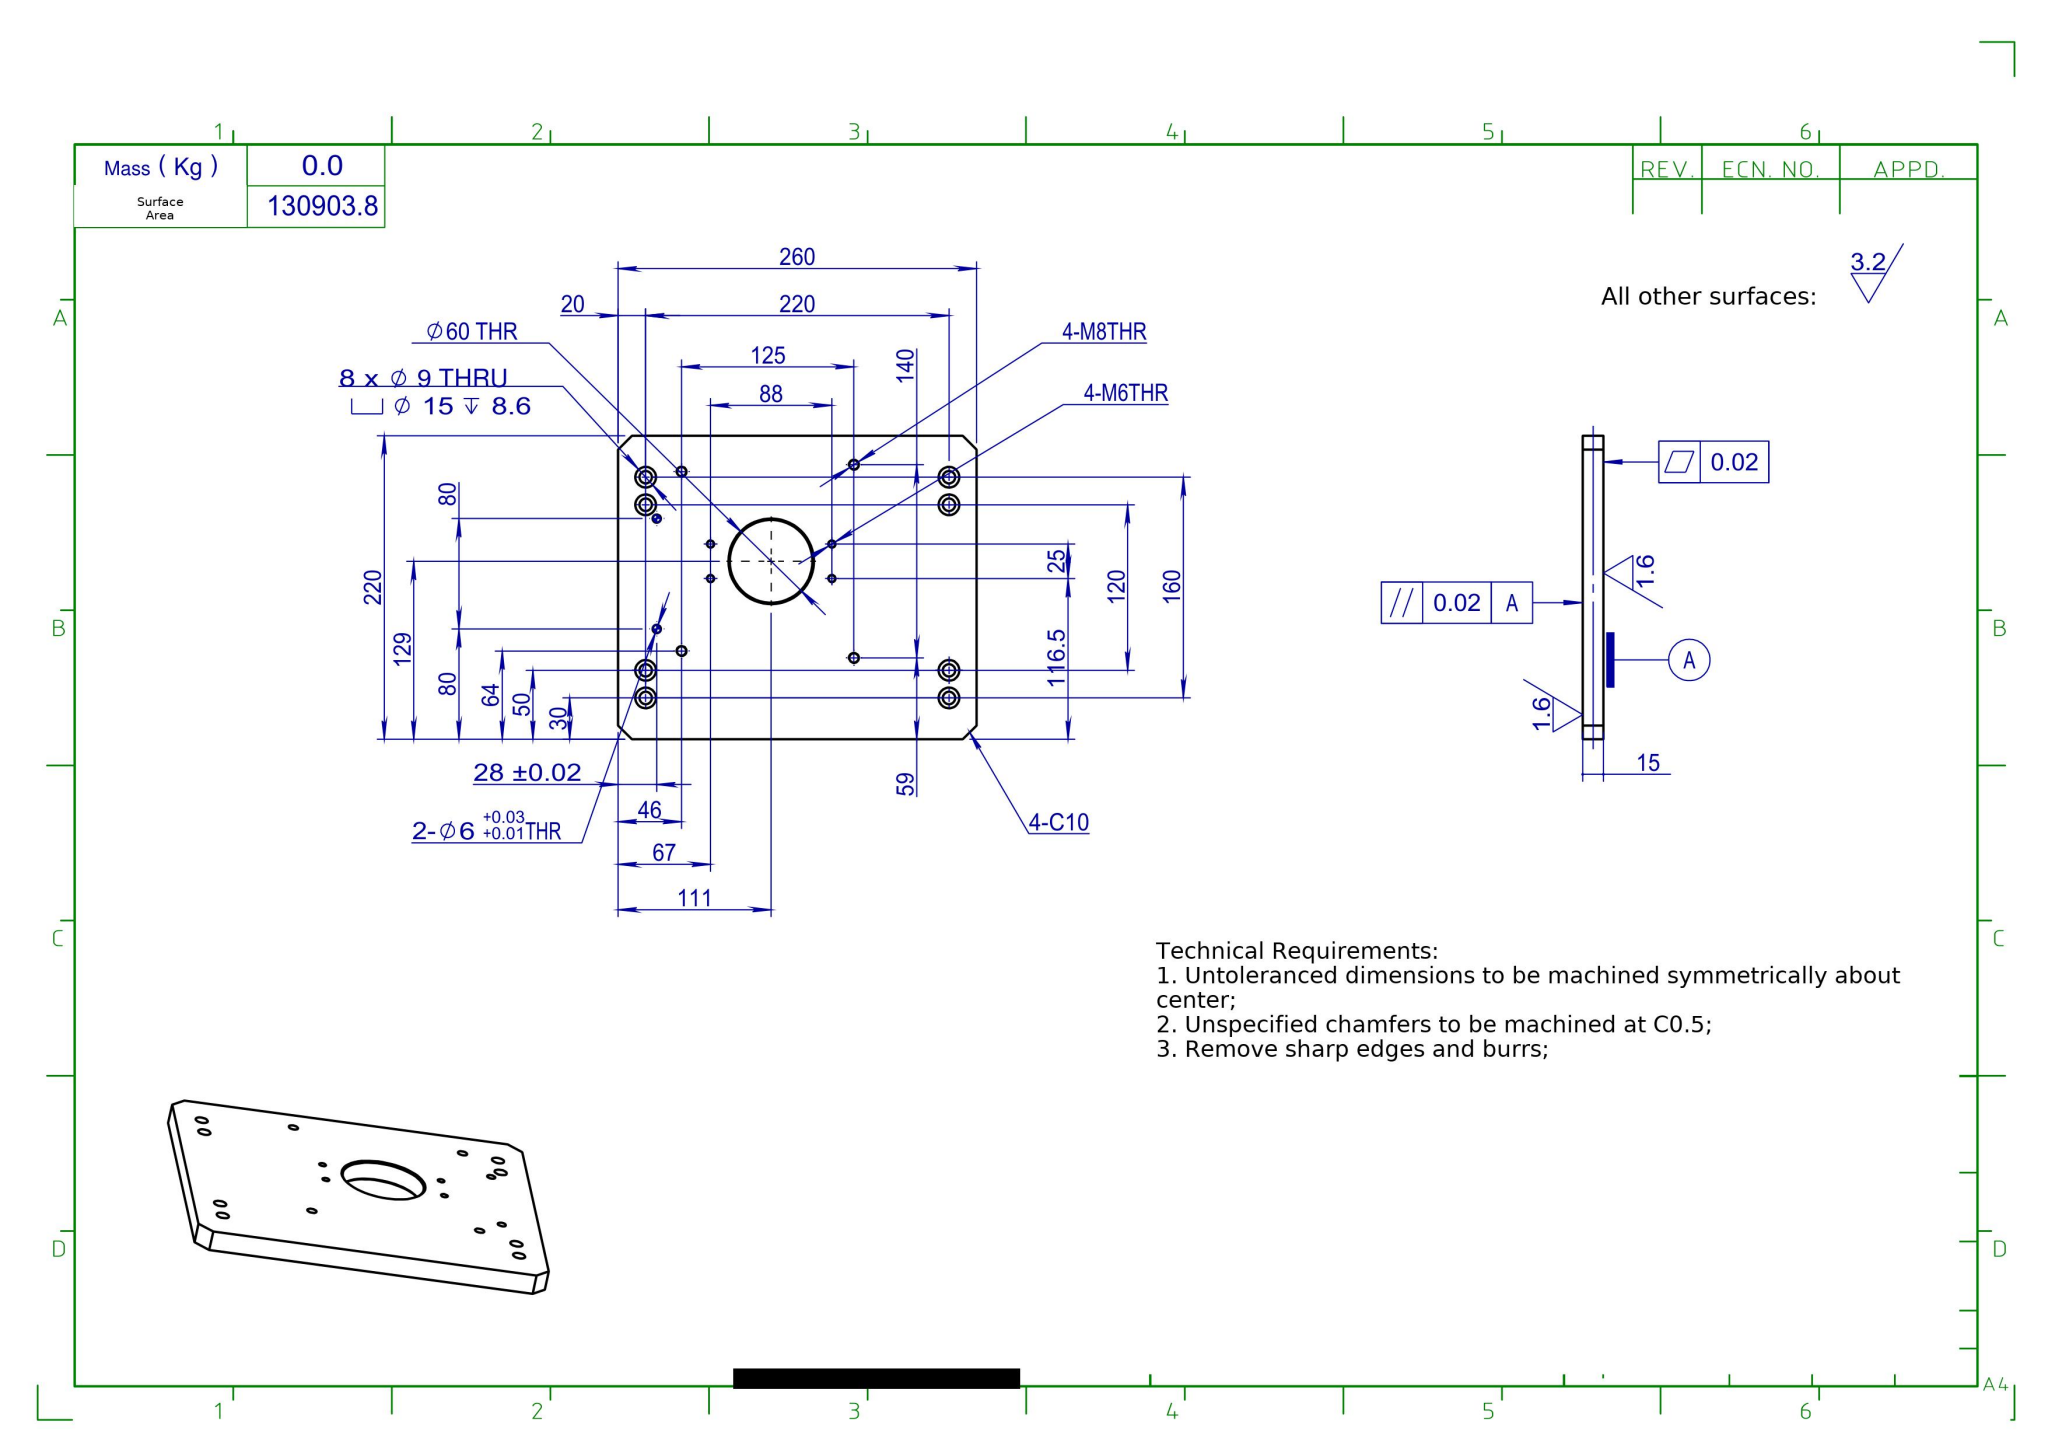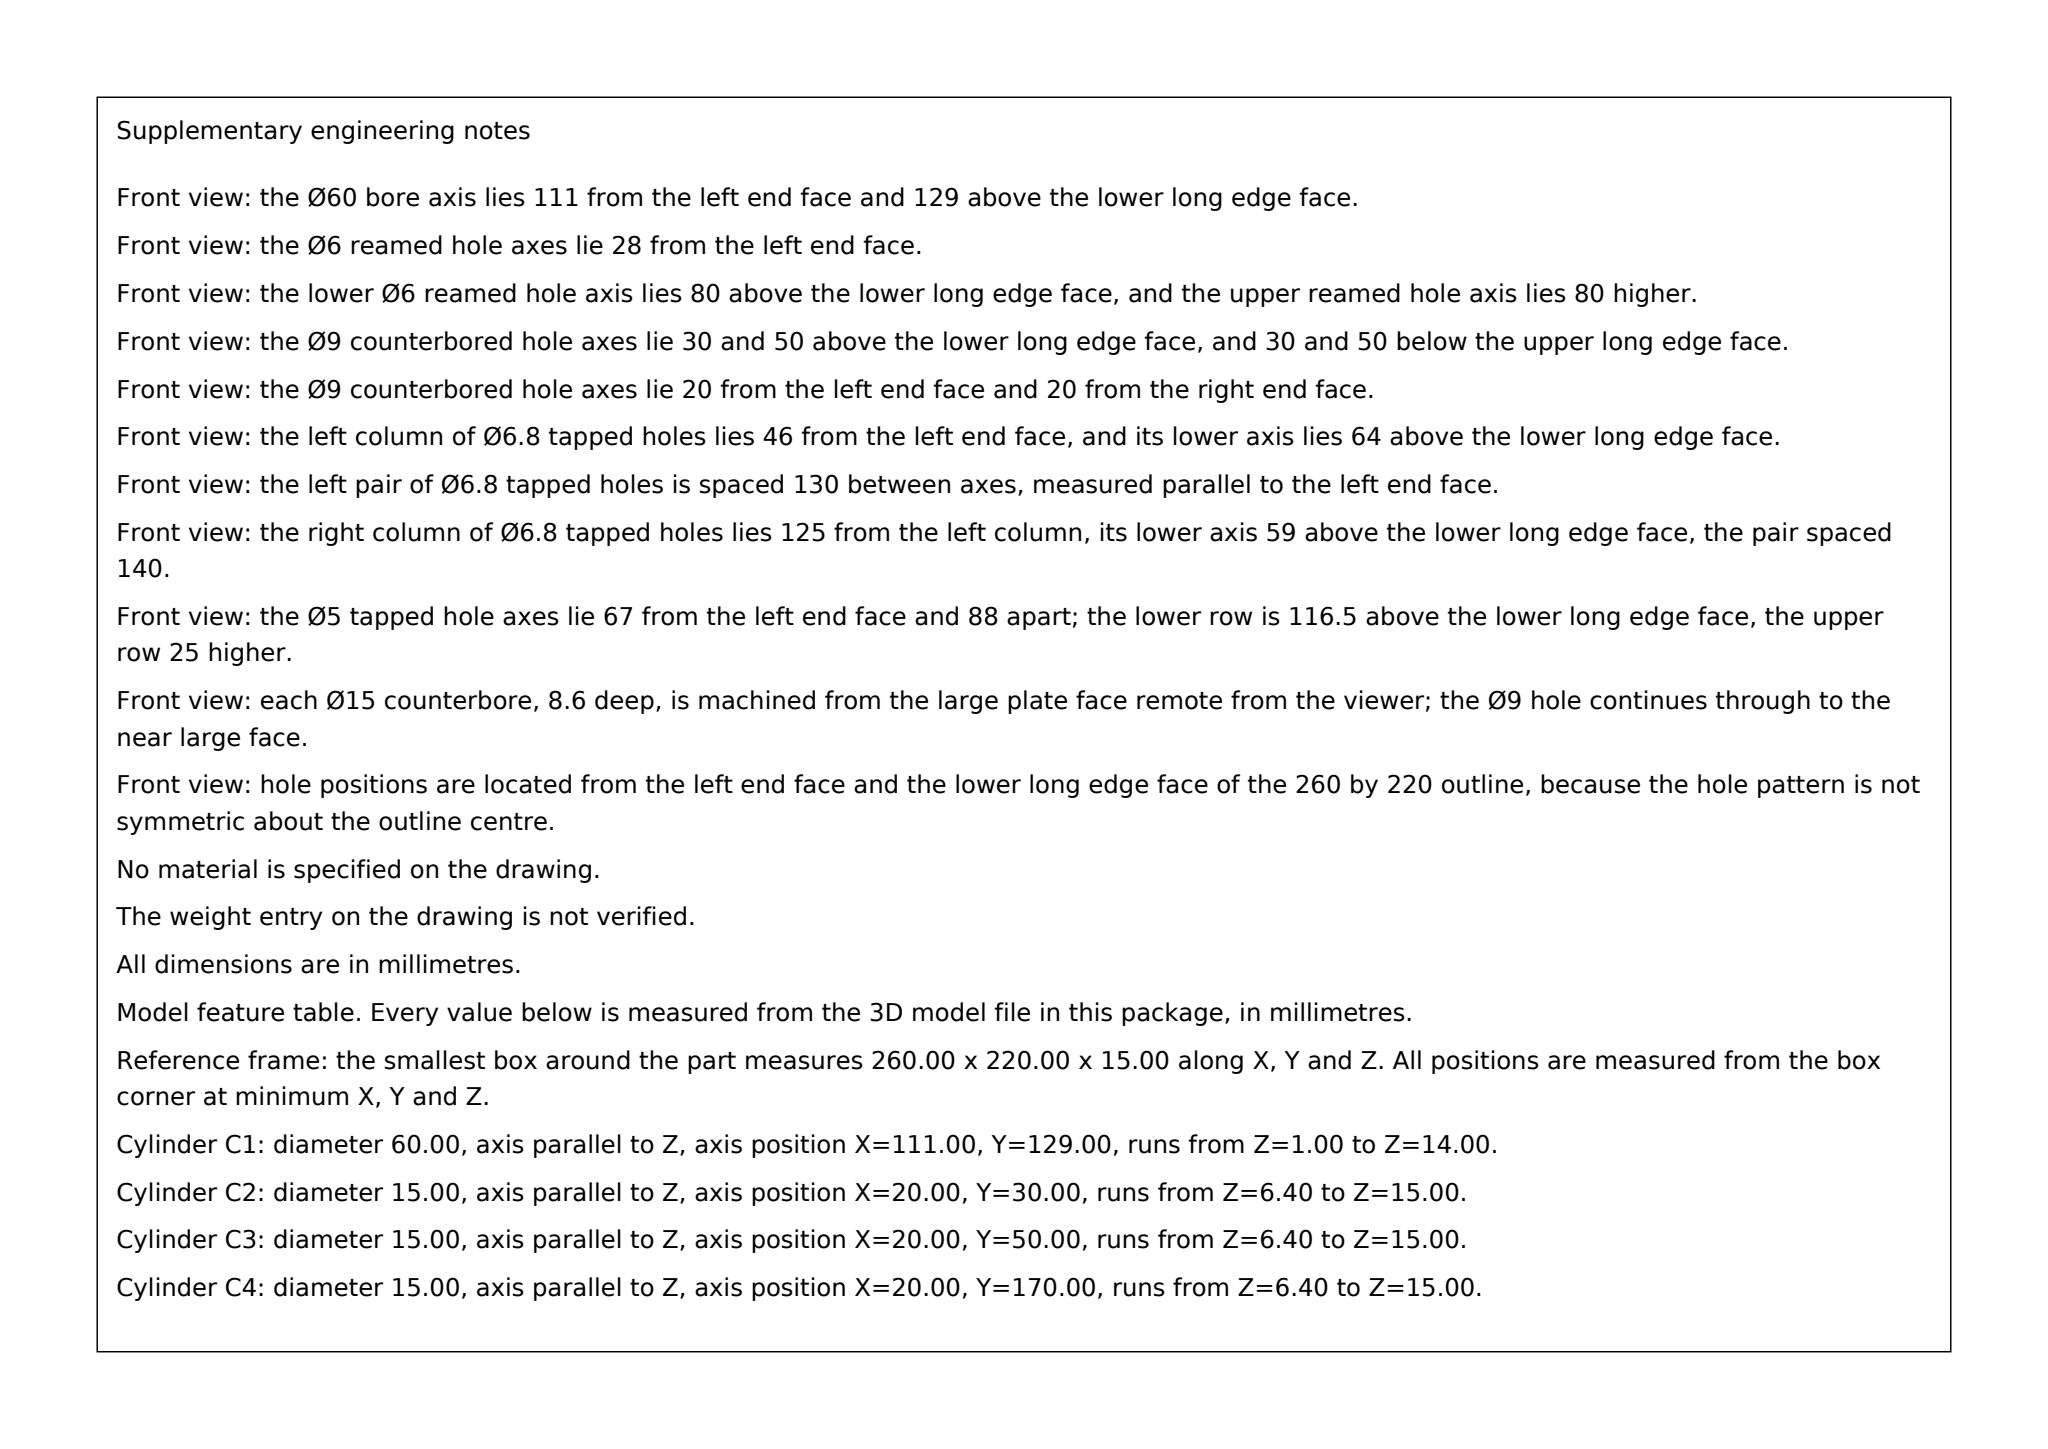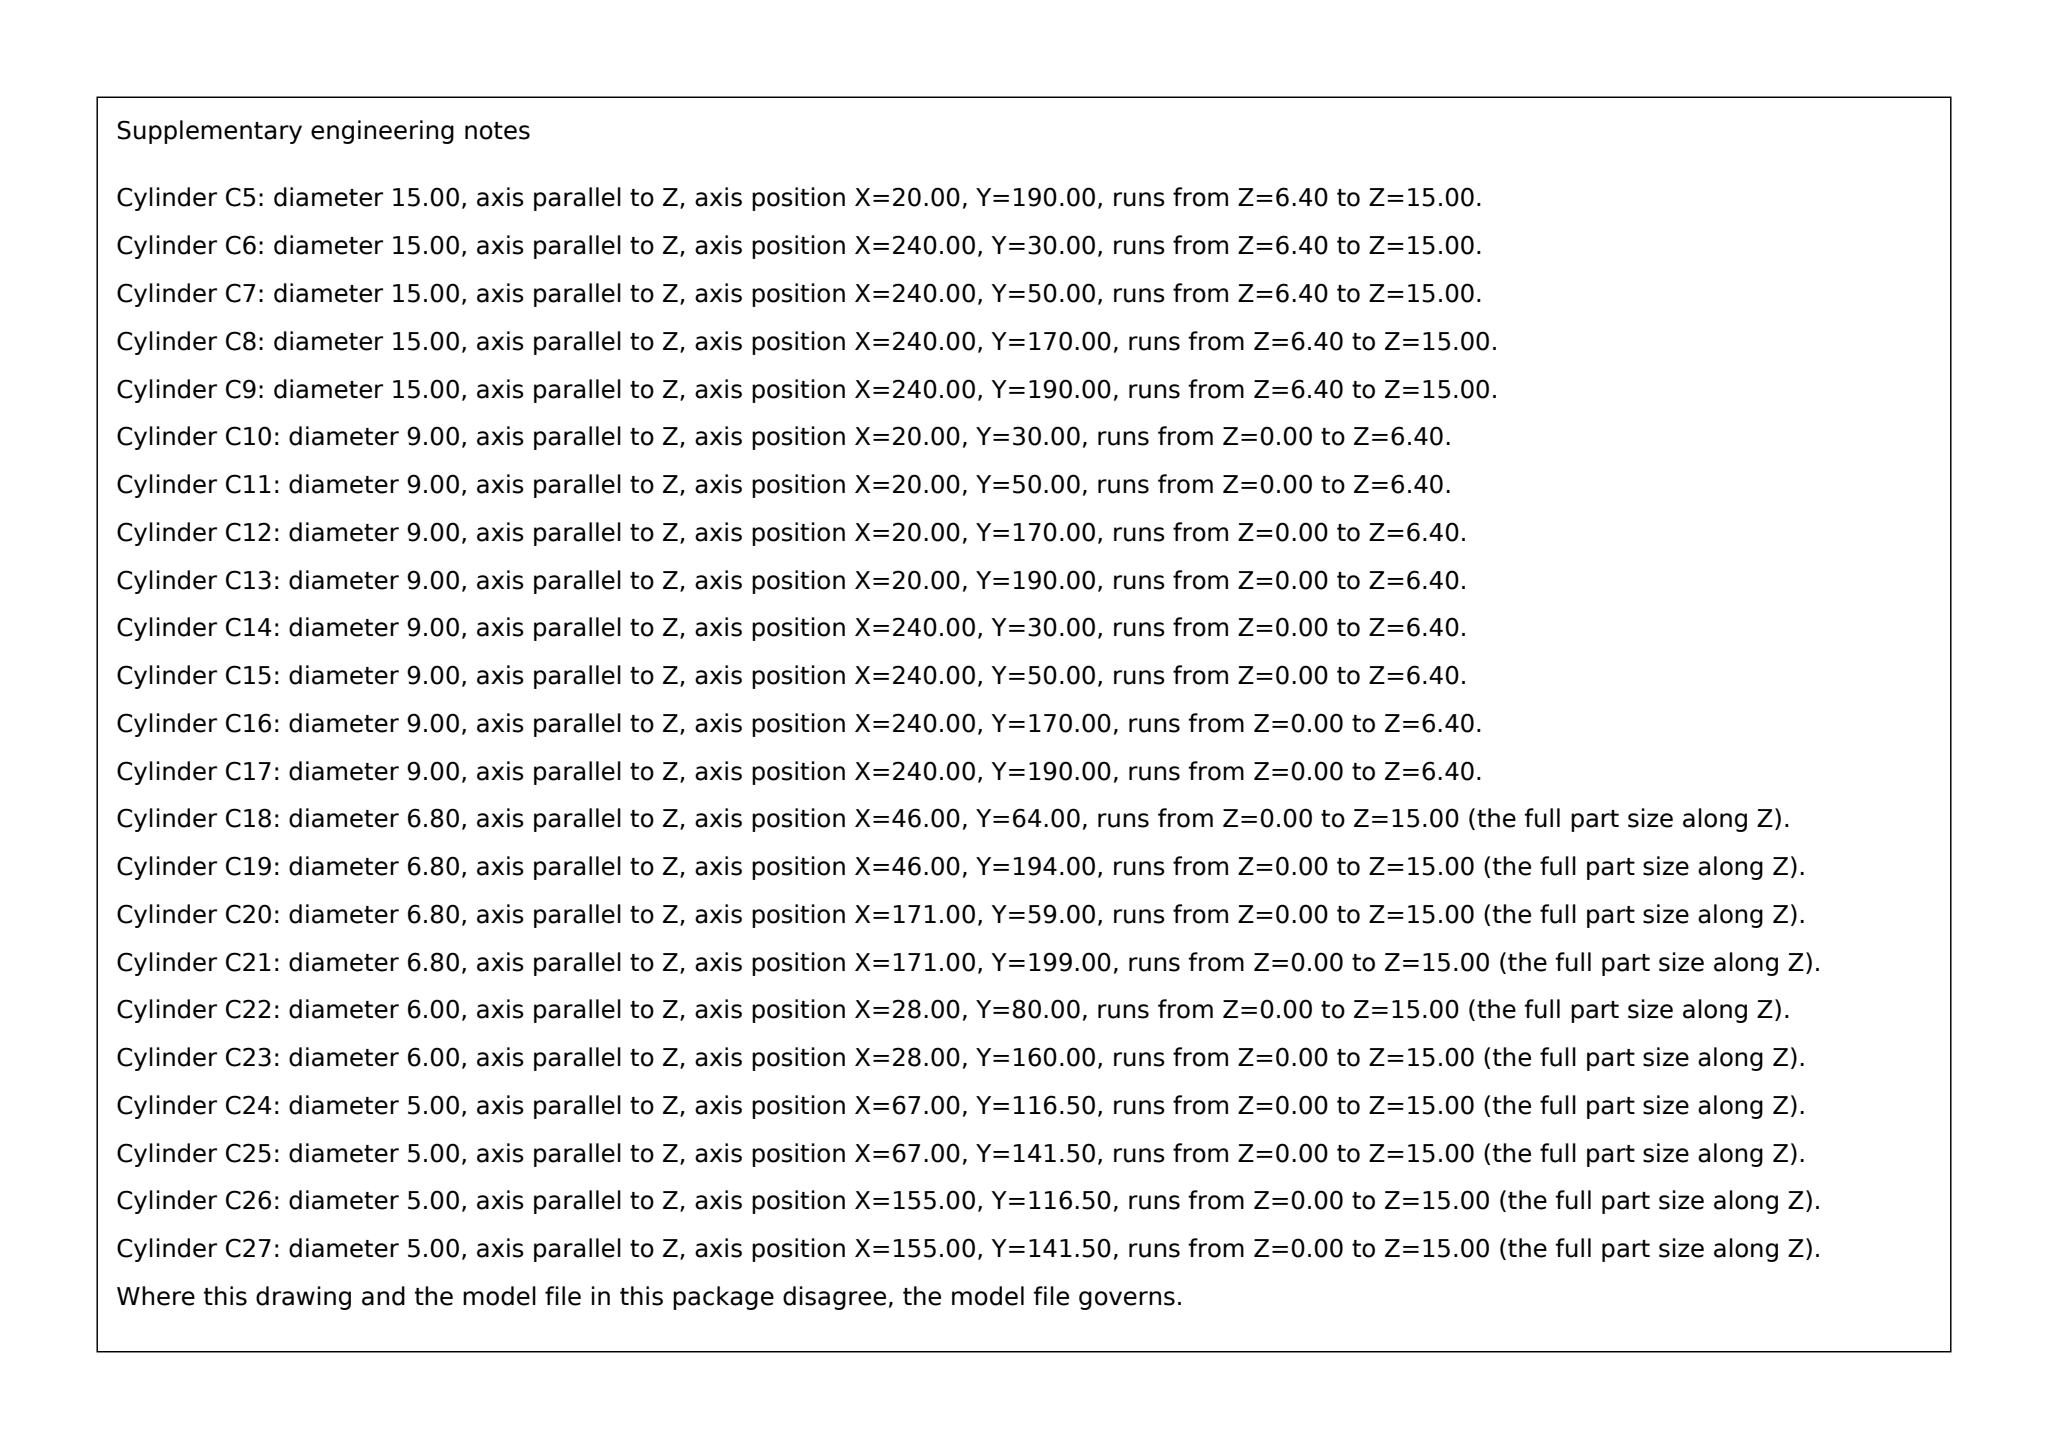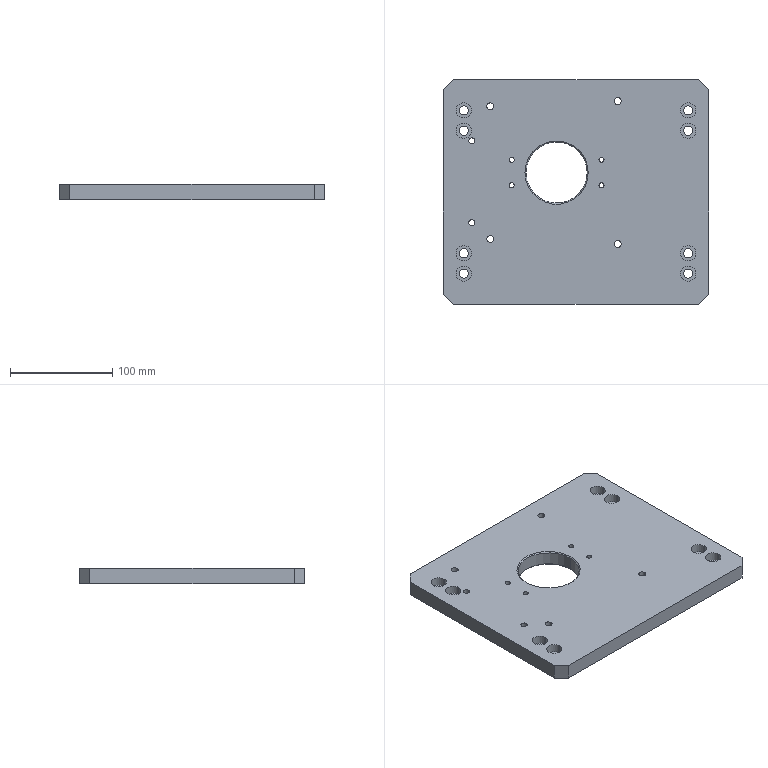Part | SolidWorks | mm | 1 solid | 76 faces | box 260 x 220 x 15 mm | volume 792777 mm3 | cylinder 54 | plane 18 | cone 4 | commonest cylinder face diameters 15 x16 9 x16 6.8 x8 5 x8 6 x4 60 x2
Drawing notes:
4-Ø5 THRU, 88 x 25 CRS, CTRD ON Ø60 BORE | from the solid: Ø5 z-cyls thru 15 at (67,116.5),(67,141.5),(155,116.5),(155,141.5); spacing 88 x 25; midpoint (111,129) = Ø60 bore ctr
Ø60 THRU BORE: CHAMFER 1 x 45° (Ø60 TO Ø62, 90° INCL) BOTH FACES | from the solid: cones[included_angle,ref_dia]: [90.0,60.0,2] and [90.0,62.0,2] on the Ø60 z-axis through bore
Ø60 THRU BORE CENTER LOCATED 111 FROM LEFT EDGE AND 129 FROM BOTTOM EDGE | from the solid: cylinders: [60.0,"z",[111.0,129.0],15.0] with bbox 260 x 220 x 15 from min corner
Ø60 THRU BORE (CTR 111 FROM LEFT EDGE, 129 FROM BOTTOM EDGE): CHAMFER 1 x 45° (Ø60 TO Ø62), BOTH FACES | from the solid: cones[included_angle,ref_dia]: [90.0,60.0,2] and [90.0,62.0,2] on the 60.0 dia z-axis cylinder at [111.0,129.0]
Ø60 THRU bore: break both ends with 1 x 45° chamfer (Ø60 to Ø62, 90° included angle). | from the solid: cones[included_angle,ref_dia]: [90.0, 60.0, 2] and [90.0, 62.0, 2] on the Ø60 z-axis through bore
Ø60 THRU bore axis located 111 from left edge (X) and 129 from bottom edge (Y) of the 260 x 220 plate. | from the solid: cylinders: [60.0, "z", [111.0, 129.0], 13.0] in 260 x 220 x 15 bbox, positions from min corner
2X Ø6 (+0.03/+0.01) REAMED THRU: X=28 FROM LEFT EDGE; Y=80 AND Y=160 FROM BOTTOM EDGE (80 APART ABOUT PLATE CENTRE Y=110? NO - AS DIMENSIONED: Y=80, Y=160). | from the solid: cylinders dia 6.0 axis z at [28.0, 80.0] and [28.0, 160.0], length 15 (THRU)
4X M8 THR (Ø6.8 TAP DRILL) IN X=46 COLUMN: Y=64 AND Y=194 FROM BOTTOM EDGE (130 HOLE-TO-HOLE SPACING). | from the solid: cylinders dia 6.8 axis z at [46.0, 64.0] and [46.0, 194.0], length 15 (THRU)
Ø60 THRU BORE AXIS: X=111 FROM LEFT EDGE, Y=129 FROM BOTTOM EDGE (replaces garbled 111/130 callout). | from the solid: cylinder dia 60.0 axis z at [111.0, 129.0]
2X Ø6 +0.03/+0.01 THRU, ON X=28 FROM LEFT EDGE; Y=80 AND Y=160 FROM BOTTOM EDGE (160 SPACING NOT SHOWN: UPPER HOLE IS 160 FROM BOTTOM EDGE / 60 FROM TOP EDGE). | from the solid: cylinders dia 6.0 axis z at [28.0, 80.0] and [28.0, 160.0], length 15 (THRU), bbox 260x220x15
4X M8 THRU (Ø6.8 TAP DRILL): TWO HOLES ON X=46 FROM LEFT EDGE AT Y=64 AND Y=194 FROM BOTTOM EDGE (130 APART); TWO HOLES ON X=171 AT Y=59 AND Y=199. | from the solid: cylinders dia 6.8 axis z at [46.0, 64.0], [46.0, 194.0], [171.0, 59.0], [171.0, 199.0], length 15 (THRU)
build123d program:
from build123d import *

# Parameters (mm, degrees)
SKETCH1_W                                            = 260
SKETCH1_H                                            = 220
EXTRUDE1_DEPTH                                       = 7.5
SKETCH2_R                                            = 30
CUT_EXTRUDE1_DEPTH                                   = 171.953
M6_TAPPED_HOLE2_D                                    = 5
CHAMFER1_SIZE                                        = 10
M8_HEX_SOCKET_HEAD_CAP_SCREW_COUNTERBORE_D           = 9
M8_HEX_SOCKET_HEAD_CAP_SCREW_COUNTERBORE_CBORE_D     = 15
M8_HEX_SOCKET_HEAD_CAP_SCREW_COUNTERBORE_CBORE_DEPTH = 8.6
M8_TAPPED_HOLE1_D                                    = 6.8
SKETCH21_R                                           = 3
CUT_EXTRUDE2_DEPTH                                   = 171.953
CHAMFER2_SIZE                                        = 1


with BuildPart() as part:
    # Sketch1 → Extrude1 (new, symmetric)
    with BuildSketch(Plane.XY):
        Rectangle(SKETCH1_W, SKETCH1_H)
    extrude(amount=EXTRUDE1_DEPTH, both=True)

    # Sketch2 → Cut-Extrude1 (cut, through all)
    with BuildSketch(Plane.XY.offset(7.5)):
        with Locations((-19, 19)):
            Circle(SKETCH2_R)
    extrude(amount=-CUT_EXTRUDE1_DEPTH, mode=Mode.SUBTRACT)

    # M6 Tapped Hole2 (through all)
    with Locations(Plane.XY.offset(7.5)):
        with Locations((-63, 31.5), (-63, 6.5), (25, 31.5), (25, 6.5)):
            Hole(M6_TAPPED_HOLE2_D / 2)

    # Chamfer1
    chamfer1_edges = [part.edges().sort_by_distance(p)[0] for p in [
        (-130, 110, 0),
        (130, 110, 0),
        (130, -110, 0),
        (-130, -110, 0),
    ]]
    chamfer(chamfer1_edges, length=CHAMFER1_SIZE)

    # M8 Hex Socket Head Cap Screw Counterbore (through all)
    with Locations(Plane.XY.offset(7.5)):
        with Locations((-110, 80), (-110, -80), (110, -80), (110, 80), (110, -60), (110, 60), (-110, 60), (-110, -60)):
            CounterBoreHole(M8_HEX_SOCKET_HEAD_CAP_SCREW_COUNTERBORE_D / 2, M8_HEX_SOCKET_HEAD_CAP_SCREW_COUNTERBORE_CBORE_D / 2, M8_HEX_SOCKET_HEAD_CAP_SCREW_COUNTERBORE_CBORE_DEPTH)

    # M8 Tapped Hole1 (through all)
    with Locations(Plane.XY.offset(7.5)):
        with Locations((-84, 84), (-84, -46), (41, -51), (41, 89)):
            Hole(M8_TAPPED_HOLE1_D / 2)

    # Sketch21 → Cut-Extrude2 (cut, through all)
    with BuildSketch(Plane.XY.offset(7.5)):
        with Locations((-102, 50)):
            Circle(SKETCH21_R)
        with Locations(Location((-102, -30, 0), (0, 0, 180))):
            Circle(SKETCH21_R)
    extrude(amount=-CUT_EXTRUDE2_DEPTH, mode=Mode.SUBTRACT)

    # Chamfer2
    chamfer2_edges = [part.edges().sort_by_distance(p)[0] for p in [
        (-49, 19, -7.5),
        (-49, 19, 7.5),
    ]]
    chamfer(chamfer2_edges, length=CHAMFER2_SIZE)


solid = part.part